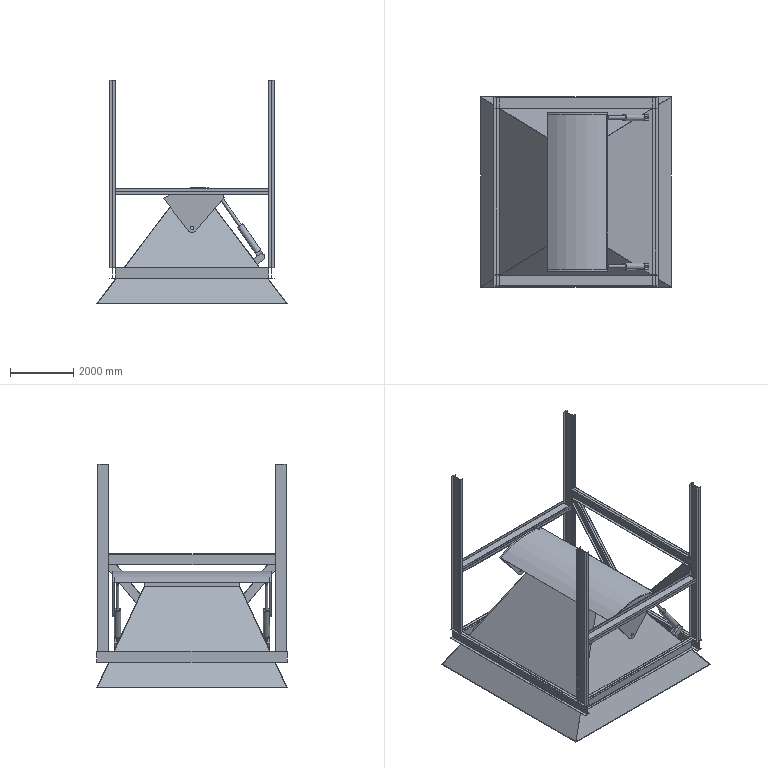Assembly | NX | mm | 17 component files | 19 solids | 290 faces | box 6000 x 6000 x 7050 mm | volume 1867179179 mm3 | plane 264 | cylinder 26 | commonest cylinder face diameters 100 x10 200 x8 400 x2 300 x2 202.237 x2 4000 x1 4032 x1
Bill of materials:
unnamed part 1 | 1 |  | Straight prismatic I/H-section member, long axis vertical, with two parallel flanges joined by a thin central web and plain square-cut ends.
unnamed part 2 | 1 |  | Long straight I/H-section member lying with its web horizontal, so the flanges stand up along both long edges; from the isometric view it looks like a shallow trough. Plain cut ends.
unnamed part 3 | 1 |  | Long straight I-section beam lying horizontally with its web vertical; equal top and bottom flanges and plain square ends.
unnamed part 4 | 1 |  | Straight prismatic I/H-section member, long axis vertical, with two flanges, a thin web and plain ends.
unnamed part 5 | 1 |  | Long straight I-section beam lying horizontally with its web vertical; the isometric view runs the opposite diagonal to parts 2 and 6. Equal flanges, plain ends.
unnamed part 6 | 2 |  | Straight I/H-section member set at an angle to the principal view axes, with flanges and a central web along its length.
unnamed part 7 | 1 |  | Long straight I-section beam lying horizontally with its web vertical; equal top and bottom flanges and plain square ends.
unnamed part 8 | 1 |  | Long straight I-section beam lying horizontally with its web vertical; equal flanges and plain ends.
unnamed part 9 | 1 |  | Long straight I-section beam lying horizontally with its web vertical; equal flanges and plain ends.
unnamed part 10 | 2 |  | Telescopic rod-and-cylinder unit: a larger-diameter cylindrical body, a smaller-diameter rod coming out of one end, and a flat rounded tab with a through-hole at each end.
unnamed part 11 | 1 |  | Straight prismatic I/H-section member, long axis vertical, with two flanges, a thin web and plain ends.
unnamed part 12 | 1 |  | Straight prismatic I/H-section member, long axis vertical, with two flanges, a thin web and plain ends.
unnamed part 13 | 1 |  | Long straight prismatic bar with an H-shaped cross-section: two parallel flat flanges joined at mid-height by a thin central web, constant section along the full length.
unnamed part 14 | 1 |  | Hollow, thin-walled shell shaped like a truncated rectangular pyramid (hood or hopper shape). The large base is open, a short rectangular collar with a rectangular through-opening sits on top, and two small cylindrical pin-like stubs stick out from the sloped outer surface.
unnamed part 15 | 1 |  | Elongated curved cover: a thin sheet curved along an arc spans the length between two flat end plates shaped like circular sectors. Each end plate narrows to a rounded tip that has one round hole. Small tab features sit at the ends, and the underside is open.
Mates:
1. touch align | zhijia_xie1 1 face | zhijia2 1 face
2. touch align | zhijia_xie1 1 face | zhijia6 1 face